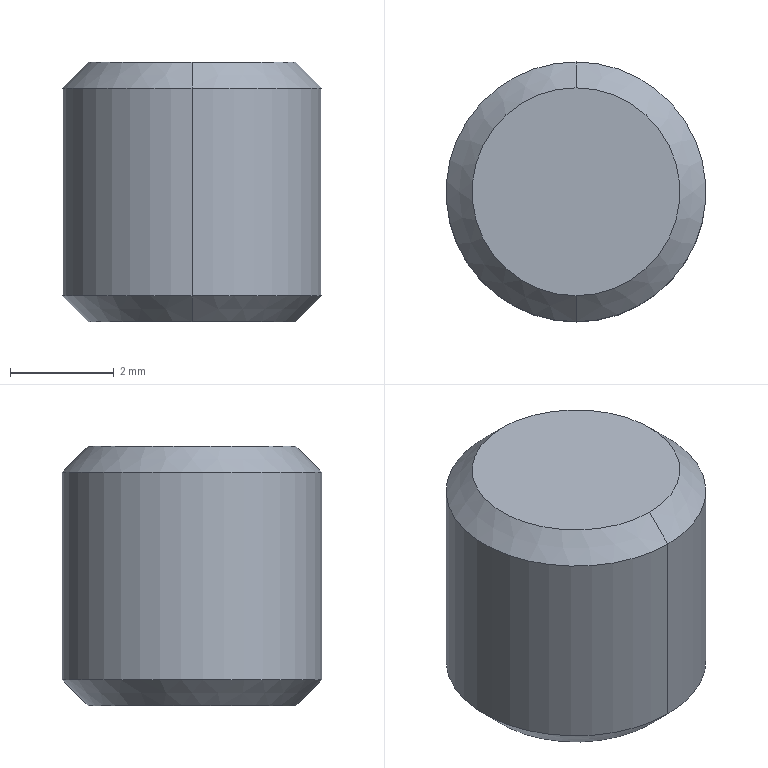Component | SolidWorks | BSH3-02-00ARubberBlankingAssembly2-1_BSH3-02-05SmallWheel-1 | 1 solid | 8 faces | box 5 x 5 x 5 mm | volume 95 mm3 | cone 4 | cylinder 2 | plane 2 | commonest cylinder face diameters 5 x2
build123d program:
from build123d import *

# Parameters (mm, degrees)
SKETCH1_R      = 2.5
EXTRUDE1_DEPTH = 5
CHAMFER1_SIZE  = 0.5


with BuildPart() as part:
    # Sketch1 → Extrude1 (new body)
    with BuildSketch(Plane.XY):
        Circle(SKETCH1_R)
    extrude(amount=EXTRUDE1_DEPTH)

    # Chamfer1
    chamfer1_edges = [part.edges().sort_by_distance(p)[0] for p in [
        (-2.5, 0, 0),
        (-2.5, 0, 5),
    ]]
    chamfer(chamfer1_edges, length=CHAMFER1_SIZE)


solid = part.part

# Placed as in the assembly
solid = solid.moved(Location((110.695, 20.762, -12.539), (0, 0, 0)))
STEP:
#1=COLOUR_RGB('',0.7922,0.8196,0.9333);
#2=FILL_AREA_STYLE_COLOUR('',#1);
#3=FILL_AREA_STYLE('',(#2));
#4=SURFACE_STYLE_FILL_AREA(#3);
#5=SURFACE_SIDE_STYLE('',(#4));
#6=SURFACE_STYLE_USAGE(.BOTH.,#5);
#7=PRESENTATION_STYLE_ASSIGNMENT((#6));
#8=CARTESIAN_POINT('',(4.358,0.8961,-0.2968));
#9=VERTEX_POINT('',#8);
#10=CARTESIAN_POINT('',(4.358,0.7386,-0.2968));
#11=VERTEX_POINT('',#10);
#12=CARTESIAN_POINT('',(4.358,0.8174,-0.2968));
#13=DIRECTION('',(0.,0.,1.));
#14=DIRECTION('',(0.,1.,0.));
#15=AXIS2_PLACEMENT_3D('',#12,#13,#14);
#16=CIRCLE('',#15,0.07874);
#17=EDGE_CURVE('',#9,#11,#16,.T.);
#18=ORIENTED_EDGE('',*,*,#17,.F.);
#19=CARTESIAN_POINT('',(4.358,0.9158,-0.3165));
#20=VERTEX_POINT('',#19);
#21=CARTESIAN_POINT('',(4.358,0.8961,-0.2968));
#22=DIRECTION('',(-0.,0.7071,-0.7071));
#23=VECTOR('',#22,39.37);
#24=LINE('',#21,#23);
#25=EDGE_CURVE('',#9,#20,#24,.T.);
#26=ORIENTED_EDGE('',*,*,#25,.T.);
#27=CARTESIAN_POINT('',(4.358,0.719,-0.3165));
#28=VERTEX_POINT('',#27);
#29=CARTESIAN_POINT('',(4.358,0.8174,-0.3165));
#30=DIRECTION('',(-0.,-0.,-1.));
#31=DIRECTION('',(0.,1.,0.));
#32=AXIS2_PLACEMENT_3D('',#29,#30,#31);
#33=CIRCLE('',#32,0.09843);
#34=EDGE_CURVE('',#28,#20,#33,.T.);
#35=ORIENTED_EDGE('',*,*,#34,.F.);
#36=CARTESIAN_POINT('',(4.358,0.7386,-0.2968));
#37=DIRECTION('',(0.,-0.7071,-0.7071));
#38=VECTOR('',#37,39.37);
#39=LINE('',#36,#38);
#40=EDGE_CURVE('',#11,#28,#39,.T.);
#41=ORIENTED_EDGE('',*,*,#40,.F.);
#42=EDGE_LOOP('',(#18,#26,#35,#41));
#43=FACE_OUTER_BOUND('',#42,.T.);
#44=CARTESIAN_POINT('',(4.358,0.8174,-0.2968));
#45=DIRECTION('',(-0.,-0.,-1.));
#46=DIRECTION('',(0.,-1.,0.));
#47=AXIS2_PLACEMENT_3D('',#44,#45,#46);
#48=CONICAL_SURFACE('',#47,0.07874,0.7854);
#49=ADVANCED_FACE('',(#43),#48,.T.);
#50=CARTESIAN_POINT('',(4.358,0.7386,-0.4937));
#51=VERTEX_POINT('',#50);
#52=CARTESIAN_POINT('',(4.358,0.8961,-0.4937));
#53=VERTEX_POINT('',#52);
#54=CARTESIAN_POINT('',(4.358,0.8174,-0.4937));
#55=DIRECTION('',(-0.,-0.,-1.));
#56=DIRECTION('',(0.,1.,0.));
#57=AXIS2_PLACEMENT_3D('',#54,#55,#56);
#58=CIRCLE('',#57,0.07874);
#59=EDGE_CURVE('',#51,#53,#58,.T.);
#60=ORIENTED_EDGE('',*,*,#59,.F.);
#61=CARTESIAN_POINT('',(4.358,0.719,-0.474));
#62=VERTEX_POINT('',#61);
#63=CARTESIAN_POINT('',(4.358,0.719,-0.474));
#64=DIRECTION('',(0.,-0.7071,0.7071));
#65=VECTOR('',#64,39.37);
#66=LINE('',#63,#65);
#67=EDGE_CURVE('',#51,#62,#66,.T.);
#68=ORIENTED_EDGE('',*,*,#67,.T.);
#69=CARTESIAN_POINT('',(4.358,0.9158,-0.474));
#70=VERTEX_POINT('',#69);
#71=CARTESIAN_POINT('',(4.358,0.8174,-0.474));
#72=DIRECTION('',(0.,0.,1.));
#73=DIRECTION('',(0.,1.,0.));
#74=AXIS2_PLACEMENT_3D('',#71,#72,#73);
#75=CIRCLE('',#74,0.09843);
#76=EDGE_CURVE('',#70,#62,#75,.T.);
#77=ORIENTED_EDGE('',*,*,#76,.F.);
#78=CARTESIAN_POINT('',(4.358,0.9158,-0.474));
#79=DIRECTION('',(-0.,0.7071,0.7071));
#80=VECTOR('',#79,39.37);
#81=LINE('',#78,#80);
#82=EDGE_CURVE('',#53,#70,#81,.T.);
#83=ORIENTED_EDGE('',*,*,#82,.F.);
#84=EDGE_LOOP('',(#60,#68,#77,#83));
#85=FACE_OUTER_BOUND('',#84,.T.);
#86=CARTESIAN_POINT('',(4.358,0.8174,-0.474));
#87=DIRECTION('',(0.,0.,1.));
#88=DIRECTION('',(0.,1.,0.));
#89=AXIS2_PLACEMENT_3D('',#86,#87,#88);
#90=CONICAL_SURFACE('',#89,0.09843,0.7854);
#91=ADVANCED_FACE('',(#85),#90,.T.);
#92=ORIENTED_EDGE('',*,*,#34,.T.);
#93=CARTESIAN_POINT('',(4.358,0.9158,-0.2968));
#94=DIRECTION('',(-0.,-0.,-1.));
#95=VECTOR('',#94,39.37);
#96=LINE('',#93,#95);
#97=EDGE_CURVE('',#20,#70,#96,.T.);
#98=ORIENTED_EDGE('',*,*,#97,.T.);
#99=ORIENTED_EDGE('',*,*,#76,.T.);
#100=CARTESIAN_POINT('',(4.358,0.719,-0.2968));
#101=DIRECTION('',(-0.,-0.,-1.));
#102=VECTOR('',#101,39.37);
#103=LINE('',#100,#102);
#104=EDGE_CURVE('',#28,#62,#103,.T.);
#105=ORIENTED_EDGE('',*,*,#104,.F.);
#106=EDGE_LOOP('',(#92,#98,#99,#105));
#107=FACE_OUTER_BOUND('',#106,.T.);
#108=CARTESIAN_POINT('',(4.358,0.8174,-0.2968));
#109=DIRECTION('',(-0.,-0.,-1.));
#110=DIRECTION('',(0.,-1.,0.));
#111=AXIS2_PLACEMENT_3D('',#108,#109,#110);
#112=CYLINDRICAL_SURFACE('',#111,0.09843);
#113=ADVANCED_FACE('',(#107),#112,.T.);
#114=ORIENTED_EDGE('',*,*,#97,.F.);
#115=CARTESIAN_POINT('',(4.358,0.8174,-0.3165));
#116=DIRECTION('',(-0.,-0.,-1.));
#117=DIRECTION('',(0.,1.,0.));
#118=AXIS2_PLACEMENT_3D('',#115,#116,#117);
#119=CIRCLE('',#118,0.09843);
#120=EDGE_CURVE('',#20,#28,#119,.T.);
#121=ORIENTED_EDGE('',*,*,#120,.T.);
#122=ORIENTED_EDGE('',*,*,#104,.T.);
#123=CARTESIAN_POINT('',(4.358,0.8174,-0.474));
#124=DIRECTION('',(0.,0.,1.));
#125=DIRECTION('',(0.,1.,0.));
#126=AXIS2_PLACEMENT_3D('',#123,#124,#125);
#127=CIRCLE('',#126,0.09843);
#128=EDGE_CURVE('',#62,#70,#127,.T.);
#129=ORIENTED_EDGE('',*,*,#128,.T.);
#130=EDGE_LOOP('',(#114,#121,#122,#129));
#131=FACE_OUTER_BOUND('',#130,.T.);
#132=CARTESIAN_POINT('',(4.358,0.8174,-0.2968));
#133=DIRECTION('',(-0.,-0.,-1.));
#134=DIRECTION('',(0.,-1.,0.));
#135=AXIS2_PLACEMENT_3D('',#132,#133,#134);
#136=CYLINDRICAL_SURFACE('',#135,0.09843);
#137=ADVANCED_FACE('',(#131),#136,.T.);
#138=CARTESIAN_POINT('',(4.358,0.8174,-0.2968));
#139=DIRECTION('',(0.,0.,1.));
#140=DIRECTION('',(0.,1.,0.));
#141=AXIS2_PLACEMENT_3D('',#138,#139,#140);
#142=CIRCLE('',#141,0.07874);
#143=EDGE_CURVE('',#11,#9,#142,.T.);
#144=ORIENTED_EDGE('',*,*,#143,.T.);
#145=ORIENTED_EDGE('',*,*,#17,.T.);
#146=EDGE_LOOP('',(#144,#145));
#147=FACE_OUTER_BOUND('',#146,.T.);
#148=CARTESIAN_POINT('',(4.358,0.8174,-0.2968));
#149=DIRECTION('',(0.,0.,1.));
#150=DIRECTION('',(-0.,1.,-0.));
#151=AXIS2_PLACEMENT_3D('',#148,#149,#150);
#152=PLANE('',#151);
#153=ADVANCED_FACE('',(#147),#152,.T.);
#154=CARTESIAN_POINT('',(4.358,0.8174,-0.4937));
#155=DIRECTION('',(-0.,-0.,-1.));
#156=DIRECTION('',(0.,1.,0.));
#157=AXIS2_PLACEMENT_3D('',#154,#155,#156);
#158=CIRCLE('',#157,0.07874);
#159=EDGE_CURVE('',#53,#51,#158,.T.);
#160=ORIENTED_EDGE('',*,*,#159,.T.);
#161=ORIENTED_EDGE('',*,*,#59,.T.);
#162=EDGE_LOOP('',(#160,#161));
#163=FACE_OUTER_BOUND('',#162,.T.);
#164=CARTESIAN_POINT('',(4.358,0.8174,-0.4937));
#165=DIRECTION('',(0.,0.,1.));
#166=DIRECTION('',(-0.,1.,-0.));
#167=AXIS2_PLACEMENT_3D('',#164,#165,#166);
#168=PLANE('',#167);
#169=ADVANCED_FACE('',(#163),#168,.F.);
#170=ORIENTED_EDGE('',*,*,#67,.F.);
#171=ORIENTED_EDGE('',*,*,#159,.F.);
#172=ORIENTED_EDGE('',*,*,#82,.T.);
#173=ORIENTED_EDGE('',*,*,#128,.F.);
#174=EDGE_LOOP('',(#170,#171,#172,#173));
#175=FACE_OUTER_BOUND('',#174,.T.);
#176=CARTESIAN_POINT('',(4.358,0.8174,-0.474));
#177=DIRECTION('',(0.,0.,1.));
#178=DIRECTION('',(0.,1.,0.));
#179=AXIS2_PLACEMENT_3D('',#176,#177,#178);
#180=CONICAL_SURFACE('',#179,0.09843,0.7854);
#181=ADVANCED_FACE('',(#175),#180,.T.);
#182=ORIENTED_EDGE('',*,*,#25,.F.);
#183=ORIENTED_EDGE('',*,*,#143,.F.);
#184=ORIENTED_EDGE('',*,*,#40,.T.);
#185=ORIENTED_EDGE('',*,*,#120,.F.);
#186=EDGE_LOOP('',(#182,#183,#184,#185));
#187=FACE_OUTER_BOUND('',#186,.T.);
#188=CARTESIAN_POINT('',(4.358,0.8174,-0.2968));
#189=DIRECTION('',(-0.,-0.,-1.));
#190=DIRECTION('',(0.,-1.,0.));
#191=AXIS2_PLACEMENT_3D('',#188,#189,#190);
#192=CONICAL_SURFACE('',#191,0.07874,0.7854);
#193=ADVANCED_FACE('',(#187),#192,.T.);
#194=CLOSED_SHELL('',(#49,#91,#113,#137,#153,#169,#181,#193));
#195=MANIFOLD_SOLID_BREP('',#194);
#196=STYLED_ITEM('',(#7),#195);
#197=PRESENTATION_LAYER_ASSIGNMENT('','',(#196));
#198=(LENGTH_UNIT()NAMED_UNIT(*)SI_UNIT($,.METRE.));
#199=LENGTH_MEASURE_WITH_UNIT(LENGTH_MEASURE(0.0254),#198);
#200=DIMENSIONAL_EXPONENTS(1.,0.,0.,0.,0.,0.,0.);
#201=(CONVERSION_BASED_UNIT('',#199)LENGTH_UNIT()NAMED_UNIT(#200));
#202=UNCERTAINTY_MEASURE_WITH_UNIT(LENGTH_MEASURE(0.00001),#201,'','');
#203=(NAMED_UNIT(*)PLANE_ANGLE_UNIT()SI_UNIT($,.RADIAN.));
#204=(NAMED_UNIT(*)SI_UNIT($,.STERADIAN.)SOLID_ANGLE_UNIT());
#205=(GEOMETRIC_REPRESENTATION_CONTEXT(3)GLOBAL_UNCERTAINTY_ASSIGNED_CONTEXT((#202))GLOBAL_UNIT_ASSIGNED_CONTEXT((#201,#203,#204))REPRESENTATION_CONTEXT('',''));
#206=MECHANICAL_DESIGN_GEOMETRIC_PRESENTATION_REPRESENTATION('',(#196),#205);
#207=CARTESIAN_POINT('',(0.,0.,0.));
#208=DIRECTION('',(0.,0.,1.));
#209=DIRECTION('',(1.,0.,0.));
#210=AXIS2_PLACEMENT_3D('',#207,#208,#209);
#211=(LENGTH_UNIT()NAMED_UNIT(*)SI_UNIT($,.METRE.));
#212=LENGTH_MEASURE_WITH_UNIT(LENGTH_MEASURE(0.0254),#211);
#213=DIMENSIONAL_EXPONENTS(1.,0.,0.,0.,0.,0.,0.);
#214=(CONVERSION_BASED_UNIT('',#212)LENGTH_UNIT()NAMED_UNIT(#213));
#215=UNCERTAINTY_MEASURE_WITH_UNIT(LENGTH_MEASURE(0.00001),#214,'','');
#216=(NAMED_UNIT(*)PLANE_ANGLE_UNIT()SI_UNIT($,.RADIAN.));
#217=(NAMED_UNIT(*)SI_UNIT($,.STERADIAN.)SOLID_ANGLE_UNIT());
#218=(GEOMETRIC_REPRESENTATION_CONTEXT(3)GLOBAL_UNCERTAINTY_ASSIGNED_CONTEXT((#215))GLOBAL_UNIT_ASSIGNED_CONTEXT((#214,#216,#217))REPRESENTATION_CONTEXT('',''));
#219=ADVANCED_BREP_SHAPE_REPRESENTATION('',(#195,#210),#218);